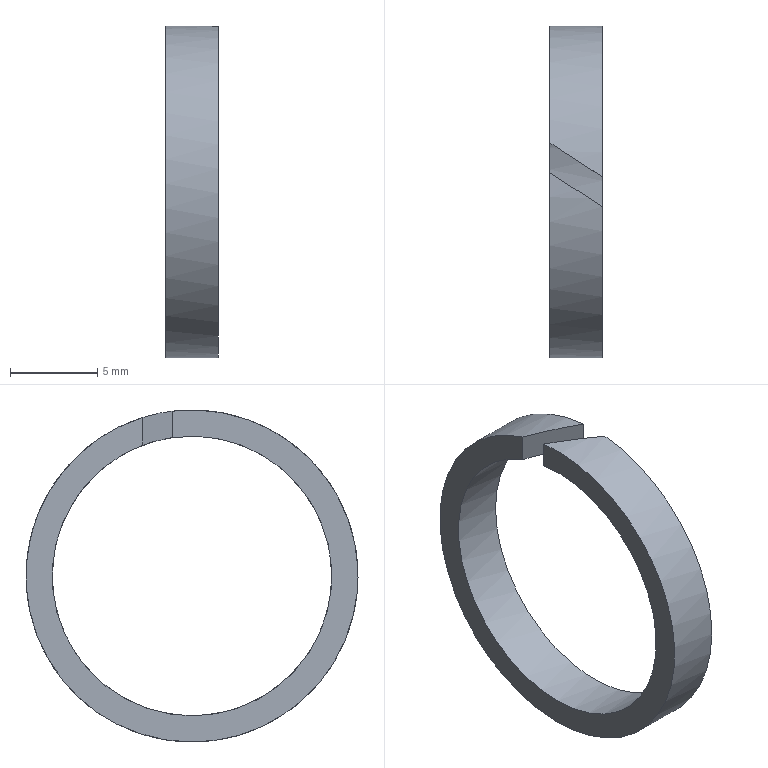Component | NX | PISTON_RING | 1 solid | 6 faces | box 3 x 19 x 19 mm | volume 240 mm3 | plane 4 | cylinder 2 | commonest cylinder face diameters 19 x1 16 x1
STEP:
#1=CARTESIAN_POINT('',(0.,0.,0.));
#2=DIRECTION('',(0.,0.,1.));
#3=DIRECTION('',(1.,0.,0.));
#4=AXIS2_PLACEMENT_3D('',#1,#2,#3);
#5=CARTESIAN_POINT('',(91.701,-35.894,50.461));
#6=VERTEX_POINT('',#5);
#7=CARTESIAN_POINT('',(88.701,-33.945,50.077));
#8=VERTEX_POINT('',#7);
#9=CARTESIAN_POINT('',(93.019,-36.75,41.));
#10=DIRECTION('',(-0.5446,-0.8387,0.));
#11=DIRECTION('',(0.8387,-0.5446,0.));
#12=AXIS2_PLACEMENT_3D('',#9,#10,#11);
#13=ELLIPSE('',#12,17.443,9.5);
#14=CARTESIAN_POINT('',(88.701,-36.75,41.));
#15=DIRECTION('',(1.,0.,0.));
#16=DIRECTION('',(0.,0.,-1.));
#17=AXIS2_PLACEMENT_3D('',#14,#15,#16);
#18=CYLINDRICAL_SURFACE('',#17,9.5);
#19=CARTESIAN_POINT('',(9.335,3.));
#20=CARTESIAN_POINT('',(9.125,-0.));
#21=B_SPLINE_CURVE_WITH_KNOTS('',1,(#19,#20),.UNSPECIFIED.,.F.,.F.,(2,2),(1.661,1.87),.PIECEWISE_BEZIER_KNOTS.);
#22=(GEOMETRIC_REPRESENTATION_CONTEXT(2)PARAMETRIC_REPRESENTATION_CONTEXT()REPRESENTATION_CONTEXT('',''));
#23=DEFINITIONAL_REPRESENTATION('',(#21),#22);
#24=PCURVE('',#18,#23);
#25=CARTESIAN_POINT('',(86.64,-32.607,53.5));
#26=DIRECTION('',(0.5446,0.8387,0.));
#27=DIRECTION('',(-0.8387,0.5446,0.));
#28=AXIS2_PLACEMENT_3D('',#25,#26,#27);
#29=PLANE('',#28);
#30=CARTESIAN_POINT('',(-25.049,-12.5));
#31=CARTESIAN_POINT('',(-25.049,3.954));
#32=CARTESIAN_POINT('',(1.115,-4.273));
#33=CARTESIAN_POINT('',(27.279,-12.5));
#34=CARTESIAN_POINT('',(1.115,-20.727));
#35=CARTESIAN_POINT('',(-25.049,-28.954));
#36=CARTESIAN_POINT('',(-25.049,-12.5));
#37=(BOUNDED_CURVE()B_SPLINE_CURVE(2,(#30,#31,#32,#33,#34,#35,#36),.UNSPECIFIED.,.T.,.F.)B_SPLINE_CURVE_WITH_KNOTS((1,2,2,2,2,1),(-2.094,0.,2.094,4.189,6.283,8.378),.UNSPECIFIED.)CURVE()GEOMETRIC_REPRESENTATION_ITEM()RATIONAL_B_SPLINE_CURVE((1.,0.5,1.,0.5,1.,0.5,1.))REPRESENTATION_ITEM(''));
#38=(GEOMETRIC_REPRESENTATION_CONTEXT(2)PARAMETRIC_REPRESENTATION_CONTEXT()REPRESENTATION_CONTEXT('',''));
#39=DEFINITIONAL_REPRESENTATION('',(#37),#38);
#40=PCURVE('',#29,#39);
#41=SURFACE_CURVE('',#13,(#24,#40),.PCURVE_S1.);
#42=EDGE_CURVE('',#6,#8,#41,.T.);
#43=ORIENTED_EDGE('',*,*,#42,.F.);
#44=CARTESIAN_POINT('',(91.701,-37.606,50.461));
#45=VERTEX_POINT('',#44);
#46=CARTESIAN_POINT('',(91.701,-36.75,41.));
#47=DIRECTION('',(1.,0.,0.));
#48=DIRECTION('',(0.,0.,1.));
#49=AXIS2_PLACEMENT_3D('',#46,#47,#48);
#50=CIRCLE('',#49,9.5);
#51=CARTESIAN_POINT('',(3.142,3.));
#52=DIRECTION('',(1.,0.));
#53=VECTOR('',#52,1.);
#54=LINE('',#51,#53);
#55=(GEOMETRIC_REPRESENTATION_CONTEXT(2)PARAMETRIC_REPRESENTATION_CONTEXT()REPRESENTATION_CONTEXT('',''));
#56=DEFINITIONAL_REPRESENTATION('',(#54),#55);
#57=PCURVE('',#18,#56);
#58=CARTESIAN_POINT('',(91.701,-36.75,41.));
#59=DIRECTION('',(1.,0.,0.));
#60=DIRECTION('',(0.,0.,-1.));
#61=AXIS2_PLACEMENT_3D('',#58,#59,#60);
#62=PLANE('',#61);
#63=CARTESIAN_POINT('',(0.,0.));
#64=DIRECTION('',(-1.,0.));
#65=AXIS2_PLACEMENT_2D('',#63,#64);
#66=CIRCLE('',#65,9.5);
#67=(GEOMETRIC_REPRESENTATION_CONTEXT(2)PARAMETRIC_REPRESENTATION_CONTEXT()REPRESENTATION_CONTEXT('',''));
#68=DEFINITIONAL_REPRESENTATION('',(#66),#67);
#69=PCURVE('',#62,#68);
#70=SURFACE_CURVE('',#50,(#57,#69),.PCURVE_S1.);
#71=EDGE_CURVE('',#45,#6,#70,.T.);
#72=ORIENTED_EDGE('',*,*,#71,.F.);
#73=CARTESIAN_POINT('',(88.701,-35.658,50.437));
#74=VERTEX_POINT('',#73);
#75=CARTESIAN_POINT('',(90.382,-36.75,41.));
#76=DIRECTION('',(0.5446,0.8387,0.));
#77=DIRECTION('',(0.8387,-0.5446,0.));
#78=AXIS2_PLACEMENT_3D('',#75,#76,#77);
#79=ELLIPSE('',#78,17.443,9.5);
#80=CARTESIAN_POINT('',(3.026,0.));
#81=CARTESIAN_POINT('',(3.232,3.));
#82=B_SPLINE_CURVE_WITH_KNOTS('',1,(#80,#81),.UNSPECIFIED.,.F.,.F.,(2,2),(4.597,4.803),.PIECEWISE_BEZIER_KNOTS.);
#83=(GEOMETRIC_REPRESENTATION_CONTEXT(2)PARAMETRIC_REPRESENTATION_CONTEXT()REPRESENTATION_CONTEXT('',''));
#84=DEFINITIONAL_REPRESENTATION('',(#82),#83);
#85=PCURVE('',#18,#84);
#86=CARTESIAN_POINT('',(96.761,-40.893,53.5));
#87=DIRECTION('',(-0.5446,-0.8387,0.));
#88=DIRECTION('',(0.8387,-0.5446,0.));
#89=AXIS2_PLACEMENT_3D('',#86,#87,#88);
#90=PLANE('',#89);
#91=CARTESIAN_POINT('',(9.837,-12.5));
#92=CARTESIAN_POINT('',(9.837,-28.954));
#93=CARTESIAN_POINT('',(-16.327,-20.727));
#94=CARTESIAN_POINT('',(-42.492,-12.5));
#95=CARTESIAN_POINT('',(-16.327,-4.273));
#96=CARTESIAN_POINT('',(9.837,3.954));
#97=CARTESIAN_POINT('',(9.837,-12.5));
#98=(BOUNDED_CURVE()B_SPLINE_CURVE(2,(#91,#92,#93,#94,#95,#96,#97),.UNSPECIFIED.,.T.,.F.)B_SPLINE_CURVE_WITH_KNOTS((1,2,2,2,2,1),(-2.094,0.,2.094,4.189,6.283,8.378),.UNSPECIFIED.)CURVE()GEOMETRIC_REPRESENTATION_ITEM()RATIONAL_B_SPLINE_CURVE((1.,0.5,1.,0.5,1.,0.5,1.))REPRESENTATION_ITEM(''));
#99=(GEOMETRIC_REPRESENTATION_CONTEXT(2)PARAMETRIC_REPRESENTATION_CONTEXT()REPRESENTATION_CONTEXT('',''));
#100=DEFINITIONAL_REPRESENTATION('',(#98),#99);
#101=PCURVE('',#90,#100);
#102=SURFACE_CURVE('',#79,(#85,#101),.PCURVE_S1.);
#103=EDGE_CURVE('',#74,#45,#102,.T.);
#104=ORIENTED_EDGE('',*,*,#103,.F.);
#105=CARTESIAN_POINT('',(88.701,-36.75,41.));
#106=DIRECTION('',(1.,0.,0.));
#107=DIRECTION('',(0.,0.,1.));
#108=AXIS2_PLACEMENT_3D('',#105,#106,#107);
#109=CIRCLE('',#108,9.5);
#110=CARTESIAN_POINT('',(-3.142,0.));
#111=DIRECTION('',(1.,0.));
#112=VECTOR('',#111,1.);
#113=LINE('',#110,#112);
#114=(GEOMETRIC_REPRESENTATION_CONTEXT(2)PARAMETRIC_REPRESENTATION_CONTEXT()REPRESENTATION_CONTEXT('',''));
#115=DEFINITIONAL_REPRESENTATION('',(#113),#114);
#116=PCURVE('',#18,#115);
#117=CARTESIAN_POINT('',(88.701,-36.75,41.));
#118=DIRECTION('',(1.,0.,0.));
#119=DIRECTION('',(0.,0.,-1.));
#120=AXIS2_PLACEMENT_3D('',#117,#118,#119);
#121=PLANE('',#120);
#122=CARTESIAN_POINT('',(0.,0.));
#123=DIRECTION('',(-1.,0.));
#124=AXIS2_PLACEMENT_2D('',#122,#123);
#125=CIRCLE('',#124,9.5);
#126=(GEOMETRIC_REPRESENTATION_CONTEXT(2)PARAMETRIC_REPRESENTATION_CONTEXT()REPRESENTATION_CONTEXT('',''));
#127=DEFINITIONAL_REPRESENTATION('',(#125),#126);
#128=PCURVE('',#121,#127);
#129=SURFACE_CURVE('',#109,(#116,#128),.PCURVE_S1.);
#130=EDGE_CURVE('',#74,#8,#129,.T.);
#131=ORIENTED_EDGE('',*,*,#130,.T.);
#132=EDGE_LOOP('',(#43,#72,#104,#131));
#133=FACE_BOUND('',#132,.T.);
#134=ADVANCED_FACE('',(#133),#18,.T.);
#135=CARTESIAN_POINT('',(88.701,-35.658,48.925));
#136=VERTEX_POINT('',#135);
#137=CARTESIAN_POINT('',(91.701,-37.606,48.954));
#138=VERTEX_POINT('',#137);
#139=CARTESIAN_POINT('',(90.382,-36.75,41.));
#140=DIRECTION('',(0.5446,0.8387,0.));
#141=DIRECTION('',(0.8387,-0.5446,0.));
#142=AXIS2_PLACEMENT_3D('',#139,#140,#141);
#143=ELLIPSE('',#142,14.689,8.);
#144=CARTESIAN_POINT('',(88.701,-36.75,41.));
#145=DIRECTION('',(1.,0.,0.));
#146=DIRECTION('',(0.,0.,-1.));
#147=AXIS2_PLACEMENT_3D('',#144,#145,#146);
#148=CYLINDRICAL_SURFACE('',#147,8.);
#149=CARTESIAN_POINT('',(3.005,0.));
#150=CARTESIAN_POINT('',(3.249,3.));
#151=B_SPLINE_CURVE_WITH_KNOTS('',1,(#149,#150),.UNSPECIFIED.,.F.,.F.,(2,2),(4.575,4.82),.PIECEWISE_BEZIER_KNOTS.);
#152=(GEOMETRIC_REPRESENTATION_CONTEXT(2)PARAMETRIC_REPRESENTATION_CONTEXT()REPRESENTATION_CONTEXT('',''));
#153=DEFINITIONAL_REPRESENTATION('',(#151),#152);
#154=PCURVE('',#148,#153);
#155=CARTESIAN_POINT('',(7.083,-12.5));
#156=CARTESIAN_POINT('',(7.083,-26.356));
#157=CARTESIAN_POINT('',(-14.95,-19.428));
#158=CARTESIAN_POINT('',(-36.983,-12.5));
#159=CARTESIAN_POINT('',(-14.95,-5.572));
#160=CARTESIAN_POINT('',(7.083,1.356));
#161=CARTESIAN_POINT('',(7.083,-12.5));
#162=(BOUNDED_CURVE()B_SPLINE_CURVE(2,(#155,#156,#157,#158,#159,#160,#161),.UNSPECIFIED.,.T.,.F.)B_SPLINE_CURVE_WITH_KNOTS((1,2,2,2,2,1),(-2.094,0.,2.094,4.189,6.283,8.378),.UNSPECIFIED.)CURVE()GEOMETRIC_REPRESENTATION_ITEM()RATIONAL_B_SPLINE_CURVE((1.,0.5,1.,0.5,1.,0.5,1.))REPRESENTATION_ITEM(''));
#163=(GEOMETRIC_REPRESENTATION_CONTEXT(2)PARAMETRIC_REPRESENTATION_CONTEXT()REPRESENTATION_CONTEXT('',''));
#164=DEFINITIONAL_REPRESENTATION('',(#162),#163);
#165=PCURVE('',#90,#164);
#166=SURFACE_CURVE('',#143,(#154,#165),.PCURVE_S1.);
#167=EDGE_CURVE('',#136,#138,#166,.T.);
#168=ORIENTED_EDGE('',*,*,#167,.F.);
#169=CARTESIAN_POINT('',(88.701,-33.945,48.492));
#170=VERTEX_POINT('',#169);
#171=CARTESIAN_POINT('',(88.701,-36.75,41.));
#172=DIRECTION('',(1.,0.,0.));
#173=DIRECTION('',(0.,0.,1.));
#174=AXIS2_PLACEMENT_3D('',#171,#172,#173);
#175=CIRCLE('',#174,8.);
#176=CARTESIAN_POINT('',(-3.142,0.));
#177=DIRECTION('',(1.,0.));
#178=VECTOR('',#177,1.);
#179=LINE('',#176,#178);
#180=(GEOMETRIC_REPRESENTATION_CONTEXT(2)PARAMETRIC_REPRESENTATION_CONTEXT()REPRESENTATION_CONTEXT('',''));
#181=DEFINITIONAL_REPRESENTATION('',(#179),#180);
#182=PCURVE('',#148,#181);
#183=CARTESIAN_POINT('',(0.,0.));
#184=DIRECTION('',(-1.,0.));
#185=AXIS2_PLACEMENT_2D('',#183,#184);
#186=CIRCLE('',#185,8.);
#187=(GEOMETRIC_REPRESENTATION_CONTEXT(2)PARAMETRIC_REPRESENTATION_CONTEXT()REPRESENTATION_CONTEXT('',''));
#188=DEFINITIONAL_REPRESENTATION('',(#186),#187);
#189=PCURVE('',#121,#188);
#190=SURFACE_CURVE('',#175,(#182,#189),.PCURVE_S1.);
#191=EDGE_CURVE('',#136,#170,#190,.T.);
#192=ORIENTED_EDGE('',*,*,#191,.T.);
#193=CARTESIAN_POINT('',(91.701,-35.894,48.954));
#194=VERTEX_POINT('',#193);
#195=CARTESIAN_POINT('',(93.019,-36.75,41.));
#196=DIRECTION('',(-0.5446,-0.8387,0.));
#197=DIRECTION('',(0.8387,-0.5446,0.));
#198=AXIS2_PLACEMENT_3D('',#195,#196,#197);
#199=ELLIPSE('',#198,14.689,8.);
#200=CARTESIAN_POINT('',(9.318,3.));
#201=CARTESIAN_POINT('',(9.067,-0.));
#202=B_SPLINE_CURVE_WITH_KNOTS('',1,(#200,#201),.UNSPECIFIED.,.F.,.F.,(2,2),(1.678,1.929),.PIECEWISE_BEZIER_KNOTS.);
#203=(GEOMETRIC_REPRESENTATION_CONTEXT(2)PARAMETRIC_REPRESENTATION_CONTEXT()REPRESENTATION_CONTEXT('',''));
#204=DEFINITIONAL_REPRESENTATION('',(#202),#203);
#205=PCURVE('',#148,#204);
#206=CARTESIAN_POINT('',(-22.295,-12.5));
#207=CARTESIAN_POINT('',(-22.295,1.356));
#208=CARTESIAN_POINT('',(-0.2617,-5.572));
#209=CARTESIAN_POINT('',(21.771,-12.5));
#210=CARTESIAN_POINT('',(-0.2617,-19.428));
#211=CARTESIAN_POINT('',(-22.295,-26.356));
#212=CARTESIAN_POINT('',(-22.295,-12.5));
#213=(BOUNDED_CURVE()B_SPLINE_CURVE(2,(#206,#207,#208,#209,#210,#211,#212),.UNSPECIFIED.,.T.,.F.)B_SPLINE_CURVE_WITH_KNOTS((1,2,2,2,2,1),(-2.094,0.,2.094,4.189,6.283,8.378),.UNSPECIFIED.)CURVE()GEOMETRIC_REPRESENTATION_ITEM()RATIONAL_B_SPLINE_CURVE((1.,0.5,1.,0.5,1.,0.5,1.))REPRESENTATION_ITEM(''));
#214=(GEOMETRIC_REPRESENTATION_CONTEXT(2)PARAMETRIC_REPRESENTATION_CONTEXT()REPRESENTATION_CONTEXT('',''));
#215=DEFINITIONAL_REPRESENTATION('',(#213),#214);
#216=PCURVE('',#29,#215);
#217=SURFACE_CURVE('',#199,(#205,#216),.PCURVE_S1.);
#218=EDGE_CURVE('',#194,#170,#217,.T.);
#219=ORIENTED_EDGE('',*,*,#218,.F.);
#220=CARTESIAN_POINT('',(91.701,-36.75,41.));
#221=DIRECTION('',(1.,0.,0.));
#222=DIRECTION('',(0.,0.,1.));
#223=AXIS2_PLACEMENT_3D('',#220,#221,#222);
#224=CIRCLE('',#223,8.);
#225=CARTESIAN_POINT('',(3.142,3.));
#226=DIRECTION('',(1.,0.));
#227=VECTOR('',#226,1.);
#228=LINE('',#225,#227);
#229=(GEOMETRIC_REPRESENTATION_CONTEXT(2)PARAMETRIC_REPRESENTATION_CONTEXT()REPRESENTATION_CONTEXT('',''));
#230=DEFINITIONAL_REPRESENTATION('',(#228),#229);
#231=PCURVE('',#148,#230);
#232=CARTESIAN_POINT('',(0.,0.));
#233=DIRECTION('',(-1.,0.));
#234=AXIS2_PLACEMENT_2D('',#232,#233);
#235=CIRCLE('',#234,8.);
#236=(GEOMETRIC_REPRESENTATION_CONTEXT(2)PARAMETRIC_REPRESENTATION_CONTEXT()REPRESENTATION_CONTEXT('',''));
#237=DEFINITIONAL_REPRESENTATION('',(#235),#236);
#238=PCURVE('',#62,#237);
#239=SURFACE_CURVE('',#224,(#231,#238),.PCURVE_S1.);
#240=EDGE_CURVE('',#138,#194,#239,.T.);
#241=ORIENTED_EDGE('',*,*,#240,.F.);
#242=EDGE_LOOP('',(#168,#192,#219,#241));
#243=FACE_BOUND('',#242,.F.);
#244=ADVANCED_FACE('',(#243),#148,.F.);
#245=ORIENTED_EDGE('',*,*,#191,.T.);
#246=CARTESIAN_POINT('',(88.701,-33.945,41.));
#247=DIRECTION('',(0.,0.,1.));
#248=VECTOR('',#247,1.);
#249=LINE('',#246,#248);
#250=CARTESIAN_POINT('',(0.,2.805));
#251=DIRECTION('',(-1.,0.));
#252=VECTOR('',#251,1.);
#253=LINE('',#250,#252);
#254=(GEOMETRIC_REPRESENTATION_CONTEXT(2)PARAMETRIC_REPRESENTATION_CONTEXT()REPRESENTATION_CONTEXT('',''));
#255=DEFINITIONAL_REPRESENTATION('',(#253),#254);
#256=PCURVE('',#121,#255);
#257=CARTESIAN_POINT('',(-2.456,-12.5));
#258=DIRECTION('',(0.,1.));
#259=VECTOR('',#258,1.);
#260=LINE('',#257,#259);
#261=(GEOMETRIC_REPRESENTATION_CONTEXT(2)PARAMETRIC_REPRESENTATION_CONTEXT()REPRESENTATION_CONTEXT('',''));
#262=DEFINITIONAL_REPRESENTATION('',(#260),#261);
#263=PCURVE('',#29,#262);
#264=SURFACE_CURVE('',#249,(#256,#263),.PCURVE_S1.);
#265=EDGE_CURVE('',#170,#8,#264,.T.);
#266=ORIENTED_EDGE('',*,*,#265,.T.);
#267=ORIENTED_EDGE('',*,*,#130,.F.);
#268=CARTESIAN_POINT('',(88.701,-35.658,41.));
#269=DIRECTION('',(0.,0.,-1.));
#270=VECTOR('',#269,1.);
#271=LINE('',#268,#270);
#272=CARTESIAN_POINT('',(0.,1.092));
#273=DIRECTION('',(1.,0.));
#274=VECTOR('',#273,1.);
#275=LINE('',#272,#274);
#276=(GEOMETRIC_REPRESENTATION_CONTEXT(2)PARAMETRIC_REPRESENTATION_CONTEXT()REPRESENTATION_CONTEXT('',''));
#277=DEFINITIONAL_REPRESENTATION('',(#275),#276);
#278=PCURVE('',#121,#277);
#279=CARTESIAN_POINT('',(-9.611,-12.5));
#280=DIRECTION('',(0.,-1.));
#281=VECTOR('',#280,1.);
#282=LINE('',#279,#281);
#283=(GEOMETRIC_REPRESENTATION_CONTEXT(2)PARAMETRIC_REPRESENTATION_CONTEXT()REPRESENTATION_CONTEXT('',''));
#284=DEFINITIONAL_REPRESENTATION('',(#282),#283);
#285=PCURVE('',#90,#284);
#286=SURFACE_CURVE('',#271,(#278,#285),.PCURVE_S1.);
#287=EDGE_CURVE('',#74,#136,#286,.T.);
#288=ORIENTED_EDGE('',*,*,#287,.T.);
#289=EDGE_LOOP('',(#245,#266,#267,#288));
#290=FACE_BOUND('',#289,.T.);
#291=ADVANCED_FACE('',(#290),#121,.F.);
#292=CARTESIAN_POINT('',(91.701,-35.894,41.));
#293=DIRECTION('',(0.,0.,1.));
#294=VECTOR('',#293,1.);
#295=LINE('',#292,#294);
#296=CARTESIAN_POINT('',(0.,0.8564));
#297=DIRECTION('',(-1.,0.));
#298=VECTOR('',#297,1.);
#299=LINE('',#296,#298);
#300=(GEOMETRIC_REPRESENTATION_CONTEXT(2)PARAMETRIC_REPRESENTATION_CONTEXT()REPRESENTATION_CONTEXT('',''));
#301=DEFINITIONAL_REPRESENTATION('',(#299),#300);
#302=PCURVE('',#62,#301);
#303=CARTESIAN_POINT('',(-6.034,-12.5));
#304=DIRECTION('',(0.,1.));
#305=VECTOR('',#304,1.);
#306=LINE('',#303,#305);
#307=(GEOMETRIC_REPRESENTATION_CONTEXT(2)PARAMETRIC_REPRESENTATION_CONTEXT()REPRESENTATION_CONTEXT('',''));
#308=DEFINITIONAL_REPRESENTATION('',(#306),#307);
#309=PCURVE('',#29,#308);
#310=SURFACE_CURVE('',#295,(#302,#309),.PCURVE_S1.);
#311=EDGE_CURVE('',#194,#6,#310,.T.);
#312=ORIENTED_EDGE('',*,*,#311,.F.);
#313=ORIENTED_EDGE('',*,*,#240,.F.);
#314=CARTESIAN_POINT('',(91.701,-37.606,41.));
#315=DIRECTION('',(0.,0.,-1.));
#316=VECTOR('',#315,1.);
#317=LINE('',#314,#316);
#318=CARTESIAN_POINT('',(0.,-0.8564));
#319=DIRECTION('',(1.,0.));
#320=VECTOR('',#319,1.);
#321=LINE('',#318,#320);
#322=(GEOMETRIC_REPRESENTATION_CONTEXT(2)PARAMETRIC_REPRESENTATION_CONTEXT()REPRESENTATION_CONTEXT('',''));
#323=DEFINITIONAL_REPRESENTATION('',(#321),#322);
#324=PCURVE('',#62,#323);
#325=CARTESIAN_POINT('',(-6.034,-12.5));
#326=DIRECTION('',(0.,-1.));
#327=VECTOR('',#326,1.);
#328=LINE('',#325,#327);
#329=(GEOMETRIC_REPRESENTATION_CONTEXT(2)PARAMETRIC_REPRESENTATION_CONTEXT()REPRESENTATION_CONTEXT('',''));
#330=DEFINITIONAL_REPRESENTATION('',(#328),#329);
#331=PCURVE('',#90,#330);
#332=SURFACE_CURVE('',#317,(#324,#331),.PCURVE_S1.);
#333=EDGE_CURVE('',#45,#138,#332,.T.);
#334=ORIENTED_EDGE('',*,*,#333,.F.);
#335=ORIENTED_EDGE('',*,*,#71,.T.);
#336=EDGE_LOOP('',(#312,#313,#334,#335));
#337=FACE_BOUND('',#336,.T.);
#338=ADVANCED_FACE('',(#337),#62,.T.);
#339=ORIENTED_EDGE('',*,*,#103,.T.);
#340=ORIENTED_EDGE('',*,*,#333,.T.);
#341=ORIENTED_EDGE('',*,*,#167,.F.);
#342=ORIENTED_EDGE('',*,*,#287,.F.);
#343=EDGE_LOOP('',(#339,#340,#341,#342));
#344=FACE_BOUND('',#343,.T.);
#345=ADVANCED_FACE('',(#344),#90,.F.);
#346=ORIENTED_EDGE('',*,*,#218,.F.);
#347=ORIENTED_EDGE('',*,*,#311,.T.);
#348=ORIENTED_EDGE('',*,*,#42,.T.);
#349=ORIENTED_EDGE('',*,*,#265,.F.);
#350=EDGE_LOOP('',(#346,#347,#348,#349));
#351=FACE_BOUND('',#350,.T.);
#352=ADVANCED_FACE('',(#351),#29,.F.);
#353=CLOSED_SHELL('',(#134,#244,#291,#338,#345,#352));
#354=MANIFOLD_SOLID_BREP('',#353);
#355=(LENGTH_UNIT()NAMED_UNIT(*)SI_UNIT(.MILLI.,.METRE.));
#356=UNCERTAINTY_MEASURE_WITH_UNIT(LENGTH_MEASURE(0.01),#355,'','');
#357=(NAMED_UNIT(*)PLANE_ANGLE_UNIT()SI_UNIT($,.RADIAN.));
#358=(NAMED_UNIT(*)SI_UNIT($,.STERADIAN.)SOLID_ANGLE_UNIT());
#359=(GEOMETRIC_REPRESENTATION_CONTEXT(3)GLOBAL_UNCERTAINTY_ASSIGNED_CONTEXT((#356))GLOBAL_UNIT_ASSIGNED_CONTEXT((#355,#357,#358))REPRESENTATION_CONTEXT('',''));
#360=ADVANCED_BREP_SHAPE_REPRESENTATION('',(#4,#354),#359);